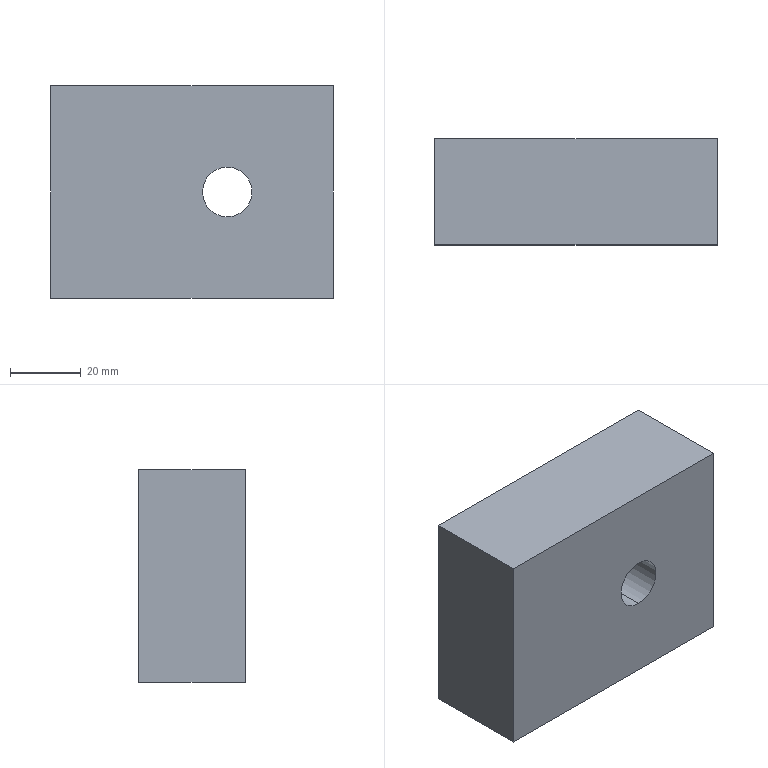Component | SolidWorks | JF21-80.1-1-3(_)-1-SOLID53-1 | 1 solid | 8 faces | box 80 x 30 x 60 mm | volume 139382 mm3 | plane 6 | cylinder 2 | commonest cylinder face diameters 14 x2
STEP:
#1=COLOUR_RGB('',0.7922,0.8196,0.9333);
#2=FILL_AREA_STYLE_COLOUR('',#1);
#3=FILL_AREA_STYLE('',(#2));
#4=SURFACE_STYLE_FILL_AREA(#3);
#5=SURFACE_SIDE_STYLE('',(#4));
#6=SURFACE_STYLE_USAGE(.BOTH.,#5);
#7=PRESENTATION_STYLE_ASSIGNMENT((#6));
#8=CARTESIAN_POINT('',(-13.78,1.961,34.921));
#9=VERTEX_POINT('',#8);
#10=CARTESIAN_POINT('',(-13.78,1.961,35.472));
#11=VERTEX_POINT('',#10);
#12=CARTESIAN_POINT('',(-13.78,1.961,35.197));
#13=DIRECTION('',(0.,1.,0.));
#14=DIRECTION('',(0.,0.,1.));
#15=AXIS2_PLACEMENT_3D('',#12,#13,#14);
#16=CIRCLE('',#15,0.2756);
#17=EDGE_CURVE('',#9,#11,#16,.T.);
#18=ORIENTED_EDGE('',*,*,#17,.F.);
#19=CARTESIAN_POINT('',(-13.78,3.142,34.921));
#20=VERTEX_POINT('',#19);
#21=CARTESIAN_POINT('',(-13.78,3.142,34.921));
#22=DIRECTION('',(0.,1.,0.));
#23=VECTOR('',#22,39.37);
#24=LINE('',#21,#23);
#25=EDGE_CURVE('',#9,#20,#24,.T.);
#26=ORIENTED_EDGE('',*,*,#25,.T.);
#27=CARTESIAN_POINT('',(-13.78,3.142,35.472));
#28=VERTEX_POINT('',#27);
#29=CARTESIAN_POINT('',(-13.78,3.142,35.197));
#30=DIRECTION('',(0.,1.,0.));
#31=DIRECTION('',(0.,0.,1.));
#32=AXIS2_PLACEMENT_3D('',#29,#30,#31);
#33=CIRCLE('',#32,0.2756);
#34=EDGE_CURVE('',#20,#28,#33,.T.);
#35=ORIENTED_EDGE('',*,*,#34,.T.);
#36=CARTESIAN_POINT('',(-13.78,3.142,35.472));
#37=DIRECTION('',(0.,1.,0.));
#38=VECTOR('',#37,39.37);
#39=LINE('',#36,#38);
#40=EDGE_CURVE('',#11,#28,#39,.T.);
#41=ORIENTED_EDGE('',*,*,#40,.F.);
#42=EDGE_LOOP('',(#18,#26,#35,#41));
#43=FACE_OUTER_BOUND('',#42,.T.);
#44=CARTESIAN_POINT('',(-13.78,3.142,35.197));
#45=DIRECTION('',(0.,1.,0.));
#46=DIRECTION('',(0.,0.,-1.));
#47=AXIS2_PLACEMENT_3D('',#44,#45,#46);
#48=CYLINDRICAL_SURFACE('',#47,0.2756);
#49=ADVANCED_FACE('',(#43),#48,.F.);
#50=CARTESIAN_POINT('',(-15.748,3.142,34.016));
#51=VERTEX_POINT('',#50);
#52=CARTESIAN_POINT('',(-15.748,3.142,36.378));
#53=VERTEX_POINT('',#52);
#54=CARTESIAN_POINT('',(-15.748,3.142,34.016));
#55=DIRECTION('',(0.,0.,1.));
#56=VECTOR('',#55,39.37);
#57=LINE('',#54,#56);
#58=EDGE_CURVE('',#51,#53,#57,.T.);
#59=ORIENTED_EDGE('',*,*,#58,.F.);
#60=CARTESIAN_POINT('',(-15.748,1.961,34.016));
#61=VERTEX_POINT('',#60);
#62=CARTESIAN_POINT('',(-15.748,1.961,34.016));
#63=DIRECTION('',(0.,1.,0.));
#64=VECTOR('',#63,39.37);
#65=LINE('',#62,#64);
#66=EDGE_CURVE('',#61,#51,#65,.T.);
#67=ORIENTED_EDGE('',*,*,#66,.F.);
#68=CARTESIAN_POINT('',(-15.748,1.961,36.378));
#69=VERTEX_POINT('',#68);
#70=CARTESIAN_POINT('',(-15.748,1.961,34.016));
#71=DIRECTION('',(0.,0.,1.));
#72=VECTOR('',#71,39.37);
#73=LINE('',#70,#72);
#74=EDGE_CURVE('',#61,#69,#73,.T.);
#75=ORIENTED_EDGE('',*,*,#74,.T.);
#76=CARTESIAN_POINT('',(-15.748,1.961,36.378));
#77=DIRECTION('',(0.,1.,0.));
#78=VECTOR('',#77,39.37);
#79=LINE('',#76,#78);
#80=EDGE_CURVE('',#69,#53,#79,.T.);
#81=ORIENTED_EDGE('',*,*,#80,.T.);
#82=EDGE_LOOP('',(#59,#67,#75,#81));
#83=FACE_OUTER_BOUND('',#82,.T.);
#84=CARTESIAN_POINT('',(-15.748,1.961,34.016));
#85=DIRECTION('',(-1.,0.,0.));
#86=DIRECTION('',(0.,0.,-1.));
#87=AXIS2_PLACEMENT_3D('',#84,#85,#86);
#88=PLANE('',#87);
#89=ADVANCED_FACE('',(#83),#88,.T.);
#90=CARTESIAN_POINT('',(-12.598,3.142,34.016));
#91=VERTEX_POINT('',#90);
#92=CARTESIAN_POINT('',(-15.748,3.142,34.016));
#93=DIRECTION('',(-1.,0.,0.));
#94=VECTOR('',#93,39.37);
#95=LINE('',#92,#94);
#96=EDGE_CURVE('',#91,#51,#95,.T.);
#97=ORIENTED_EDGE('',*,*,#96,.F.);
#98=CARTESIAN_POINT('',(-12.598,1.961,34.016));
#99=VERTEX_POINT('',#98);
#100=CARTESIAN_POINT('',(-12.598,1.961,34.016));
#101=DIRECTION('',(0.,1.,0.));
#102=VECTOR('',#101,39.37);
#103=LINE('',#100,#102);
#104=EDGE_CURVE('',#99,#91,#103,.T.);
#105=ORIENTED_EDGE('',*,*,#104,.F.);
#106=CARTESIAN_POINT('',(-15.748,1.961,34.016));
#107=DIRECTION('',(-1.,0.,0.));
#108=VECTOR('',#107,39.37);
#109=LINE('',#106,#108);
#110=EDGE_CURVE('',#99,#61,#109,.T.);
#111=ORIENTED_EDGE('',*,*,#110,.T.);
#112=ORIENTED_EDGE('',*,*,#66,.T.);
#113=EDGE_LOOP('',(#97,#105,#111,#112));
#114=FACE_OUTER_BOUND('',#113,.T.);
#115=CARTESIAN_POINT('',(-15.748,1.961,34.016));
#116=DIRECTION('',(0.,0.,-1.));
#117=DIRECTION('',(1.,0.,0.));
#118=AXIS2_PLACEMENT_3D('',#115,#116,#117);
#119=PLANE('',#118);
#120=ADVANCED_FACE('',(#114),#119,.T.);
#121=CARTESIAN_POINT('',(-12.598,3.142,36.378));
#122=VERTEX_POINT('',#121);
#123=CARTESIAN_POINT('',(-12.598,3.142,34.016));
#124=DIRECTION('',(0.,0.,-1.));
#125=VECTOR('',#124,39.37);
#126=LINE('',#123,#125);
#127=EDGE_CURVE('',#122,#91,#126,.T.);
#128=ORIENTED_EDGE('',*,*,#127,.F.);
#129=CARTESIAN_POINT('',(-12.598,1.961,36.378));
#130=VERTEX_POINT('',#129);
#131=CARTESIAN_POINT('',(-12.598,1.961,36.378));
#132=DIRECTION('',(0.,1.,0.));
#133=VECTOR('',#132,39.37);
#134=LINE('',#131,#133);
#135=EDGE_CURVE('',#130,#122,#134,.T.);
#136=ORIENTED_EDGE('',*,*,#135,.F.);
#137=CARTESIAN_POINT('',(-12.598,1.961,34.016));
#138=DIRECTION('',(0.,0.,-1.));
#139=VECTOR('',#138,39.37);
#140=LINE('',#137,#139);
#141=EDGE_CURVE('',#130,#99,#140,.T.);
#142=ORIENTED_EDGE('',*,*,#141,.T.);
#143=ORIENTED_EDGE('',*,*,#104,.T.);
#144=EDGE_LOOP('',(#128,#136,#142,#143));
#145=FACE_OUTER_BOUND('',#144,.T.);
#146=CARTESIAN_POINT('',(-12.598,1.961,34.016));
#147=DIRECTION('',(1.,0.,0.));
#148=DIRECTION('',(0.,0.,1.));
#149=AXIS2_PLACEMENT_3D('',#146,#147,#148);
#150=PLANE('',#149);
#151=ADVANCED_FACE('',(#145),#150,.T.);
#152=CARTESIAN_POINT('',(-15.748,3.142,36.378));
#153=DIRECTION('',(1.,0.,0.));
#154=VECTOR('',#153,39.37);
#155=LINE('',#152,#154);
#156=EDGE_CURVE('',#53,#122,#155,.T.);
#157=ORIENTED_EDGE('',*,*,#156,.F.);
#158=ORIENTED_EDGE('',*,*,#80,.F.);
#159=CARTESIAN_POINT('',(-15.748,1.961,36.378));
#160=DIRECTION('',(1.,0.,0.));
#161=VECTOR('',#160,39.37);
#162=LINE('',#159,#161);
#163=EDGE_CURVE('',#69,#130,#162,.T.);
#164=ORIENTED_EDGE('',*,*,#163,.T.);
#165=ORIENTED_EDGE('',*,*,#135,.T.);
#166=EDGE_LOOP('',(#157,#158,#164,#165));
#167=FACE_OUTER_BOUND('',#166,.T.);
#168=CARTESIAN_POINT('',(-15.748,1.961,36.378));
#169=DIRECTION('',(0.,0.,1.));
#170=DIRECTION('',(-1.,0.,0.));
#171=AXIS2_PLACEMENT_3D('',#168,#169,#170);
#172=PLANE('',#171);
#173=ADVANCED_FACE('',(#167),#172,.T.);
#174=CARTESIAN_POINT('',(-13.78,1.961,35.197));
#175=DIRECTION('',(0.,1.,0.));
#176=DIRECTION('',(0.,0.,1.));
#177=AXIS2_PLACEMENT_3D('',#174,#175,#176);
#178=CIRCLE('',#177,0.2756);
#179=EDGE_CURVE('',#11,#9,#178,.T.);
#180=ORIENTED_EDGE('',*,*,#179,.T.);
#181=ORIENTED_EDGE('',*,*,#17,.T.);
#182=EDGE_LOOP('',(#180,#181));
#183=FACE_BOUND('',#182,.T.);
#184=ORIENTED_EDGE('',*,*,#74,.F.);
#185=ORIENTED_EDGE('',*,*,#110,.F.);
#186=ORIENTED_EDGE('',*,*,#141,.F.);
#187=ORIENTED_EDGE('',*,*,#163,.F.);
#188=EDGE_LOOP('',(#184,#185,#186,#187));
#189=FACE_OUTER_BOUND('',#188,.T.);
#190=CARTESIAN_POINT('',(-15.748,1.961,36.378));
#191=DIRECTION('',(0.,1.,0.));
#192=DIRECTION('',(0.,0.,-1.));
#193=AXIS2_PLACEMENT_3D('',#190,#191,#192);
#194=PLANE('',#193);
#195=ADVANCED_FACE('',(#183,#189),#194,.F.);
#196=CARTESIAN_POINT('',(-13.78,3.142,35.197));
#197=DIRECTION('',(0.,1.,0.));
#198=DIRECTION('',(0.,0.,1.));
#199=AXIS2_PLACEMENT_3D('',#196,#197,#198);
#200=CIRCLE('',#199,0.2756);
#201=EDGE_CURVE('',#28,#20,#200,.T.);
#202=ORIENTED_EDGE('',*,*,#201,.F.);
#203=ORIENTED_EDGE('',*,*,#34,.F.);
#204=EDGE_LOOP('',(#202,#203));
#205=FACE_BOUND('',#204,.T.);
#206=ORIENTED_EDGE('',*,*,#58,.T.);
#207=ORIENTED_EDGE('',*,*,#156,.T.);
#208=ORIENTED_EDGE('',*,*,#127,.T.);
#209=ORIENTED_EDGE('',*,*,#96,.T.);
#210=EDGE_LOOP('',(#206,#207,#208,#209));
#211=FACE_OUTER_BOUND('',#210,.T.);
#212=CARTESIAN_POINT('',(-15.748,3.142,36.378));
#213=DIRECTION('',(0.,1.,0.));
#214=DIRECTION('',(0.,0.,-1.));
#215=AXIS2_PLACEMENT_3D('',#212,#213,#214);
#216=PLANE('',#215);
#217=ADVANCED_FACE('',(#205,#211),#216,.T.);
#218=ORIENTED_EDGE('',*,*,#25,.F.);
#219=ORIENTED_EDGE('',*,*,#179,.F.);
#220=ORIENTED_EDGE('',*,*,#40,.T.);
#221=ORIENTED_EDGE('',*,*,#201,.T.);
#222=EDGE_LOOP('',(#218,#219,#220,#221));
#223=FACE_OUTER_BOUND('',#222,.T.);
#224=CARTESIAN_POINT('',(-13.78,3.142,35.197));
#225=DIRECTION('',(0.,1.,0.));
#226=DIRECTION('',(0.,0.,-1.));
#227=AXIS2_PLACEMENT_3D('',#224,#225,#226);
#228=CYLINDRICAL_SURFACE('',#227,0.2756);
#229=ADVANCED_FACE('',(#223),#228,.F.);
#230=CLOSED_SHELL('',(#49,#89,#120,#151,#173,#195,#217,#229));
#231=MANIFOLD_SOLID_BREP('',#230);
#232=STYLED_ITEM('',(#7),#231);
#233=(LENGTH_UNIT()NAMED_UNIT(*)SI_UNIT($,.METRE.));
#234=LENGTH_MEASURE_WITH_UNIT(LENGTH_MEASURE(0.0254),#233);
#235=DIMENSIONAL_EXPONENTS(1.,0.,0.,0.,0.,0.,0.);
#236=(CONVERSION_BASED_UNIT('',#234)LENGTH_UNIT()NAMED_UNIT(#235));
#237=UNCERTAINTY_MEASURE_WITH_UNIT(LENGTH_MEASURE(0.00001),#236,'','');
#238=(NAMED_UNIT(*)PLANE_ANGLE_UNIT()SI_UNIT($,.RADIAN.));
#239=(NAMED_UNIT(*)SI_UNIT($,.STERADIAN.)SOLID_ANGLE_UNIT());
#240=(GEOMETRIC_REPRESENTATION_CONTEXT(3)GLOBAL_UNCERTAINTY_ASSIGNED_CONTEXT((#237))GLOBAL_UNIT_ASSIGNED_CONTEXT((#236,#238,#239))REPRESENTATION_CONTEXT('',''));
#241=MECHANICAL_DESIGN_GEOMETRIC_PRESENTATION_REPRESENTATION('',(#232),#240);
#242=CARTESIAN_POINT('',(0.,0.,0.));
#243=DIRECTION('',(0.,0.,1.));
#244=DIRECTION('',(1.,0.,0.));
#245=AXIS2_PLACEMENT_3D('',#242,#243,#244);
#246=(LENGTH_UNIT()NAMED_UNIT(*)SI_UNIT($,.METRE.));
#247=LENGTH_MEASURE_WITH_UNIT(LENGTH_MEASURE(0.0254),#246);
#248=DIMENSIONAL_EXPONENTS(1.,0.,0.,0.,0.,0.,0.);
#249=(CONVERSION_BASED_UNIT('',#247)LENGTH_UNIT()NAMED_UNIT(#248));
#250=UNCERTAINTY_MEASURE_WITH_UNIT(LENGTH_MEASURE(0.00001),#249,'','');
#251=(NAMED_UNIT(*)PLANE_ANGLE_UNIT()SI_UNIT($,.RADIAN.));
#252=(NAMED_UNIT(*)SI_UNIT($,.STERADIAN.)SOLID_ANGLE_UNIT());
#253=(GEOMETRIC_REPRESENTATION_CONTEXT(3)GLOBAL_UNCERTAINTY_ASSIGNED_CONTEXT((#250))GLOBAL_UNIT_ASSIGNED_CONTEXT((#249,#251,#252))REPRESENTATION_CONTEXT('',''));
#254=ADVANCED_BREP_SHAPE_REPRESENTATION('',(#231,#245),#253);
#255=PRESENTATION_LAYER_ASSIGNMENT('','',(#232));